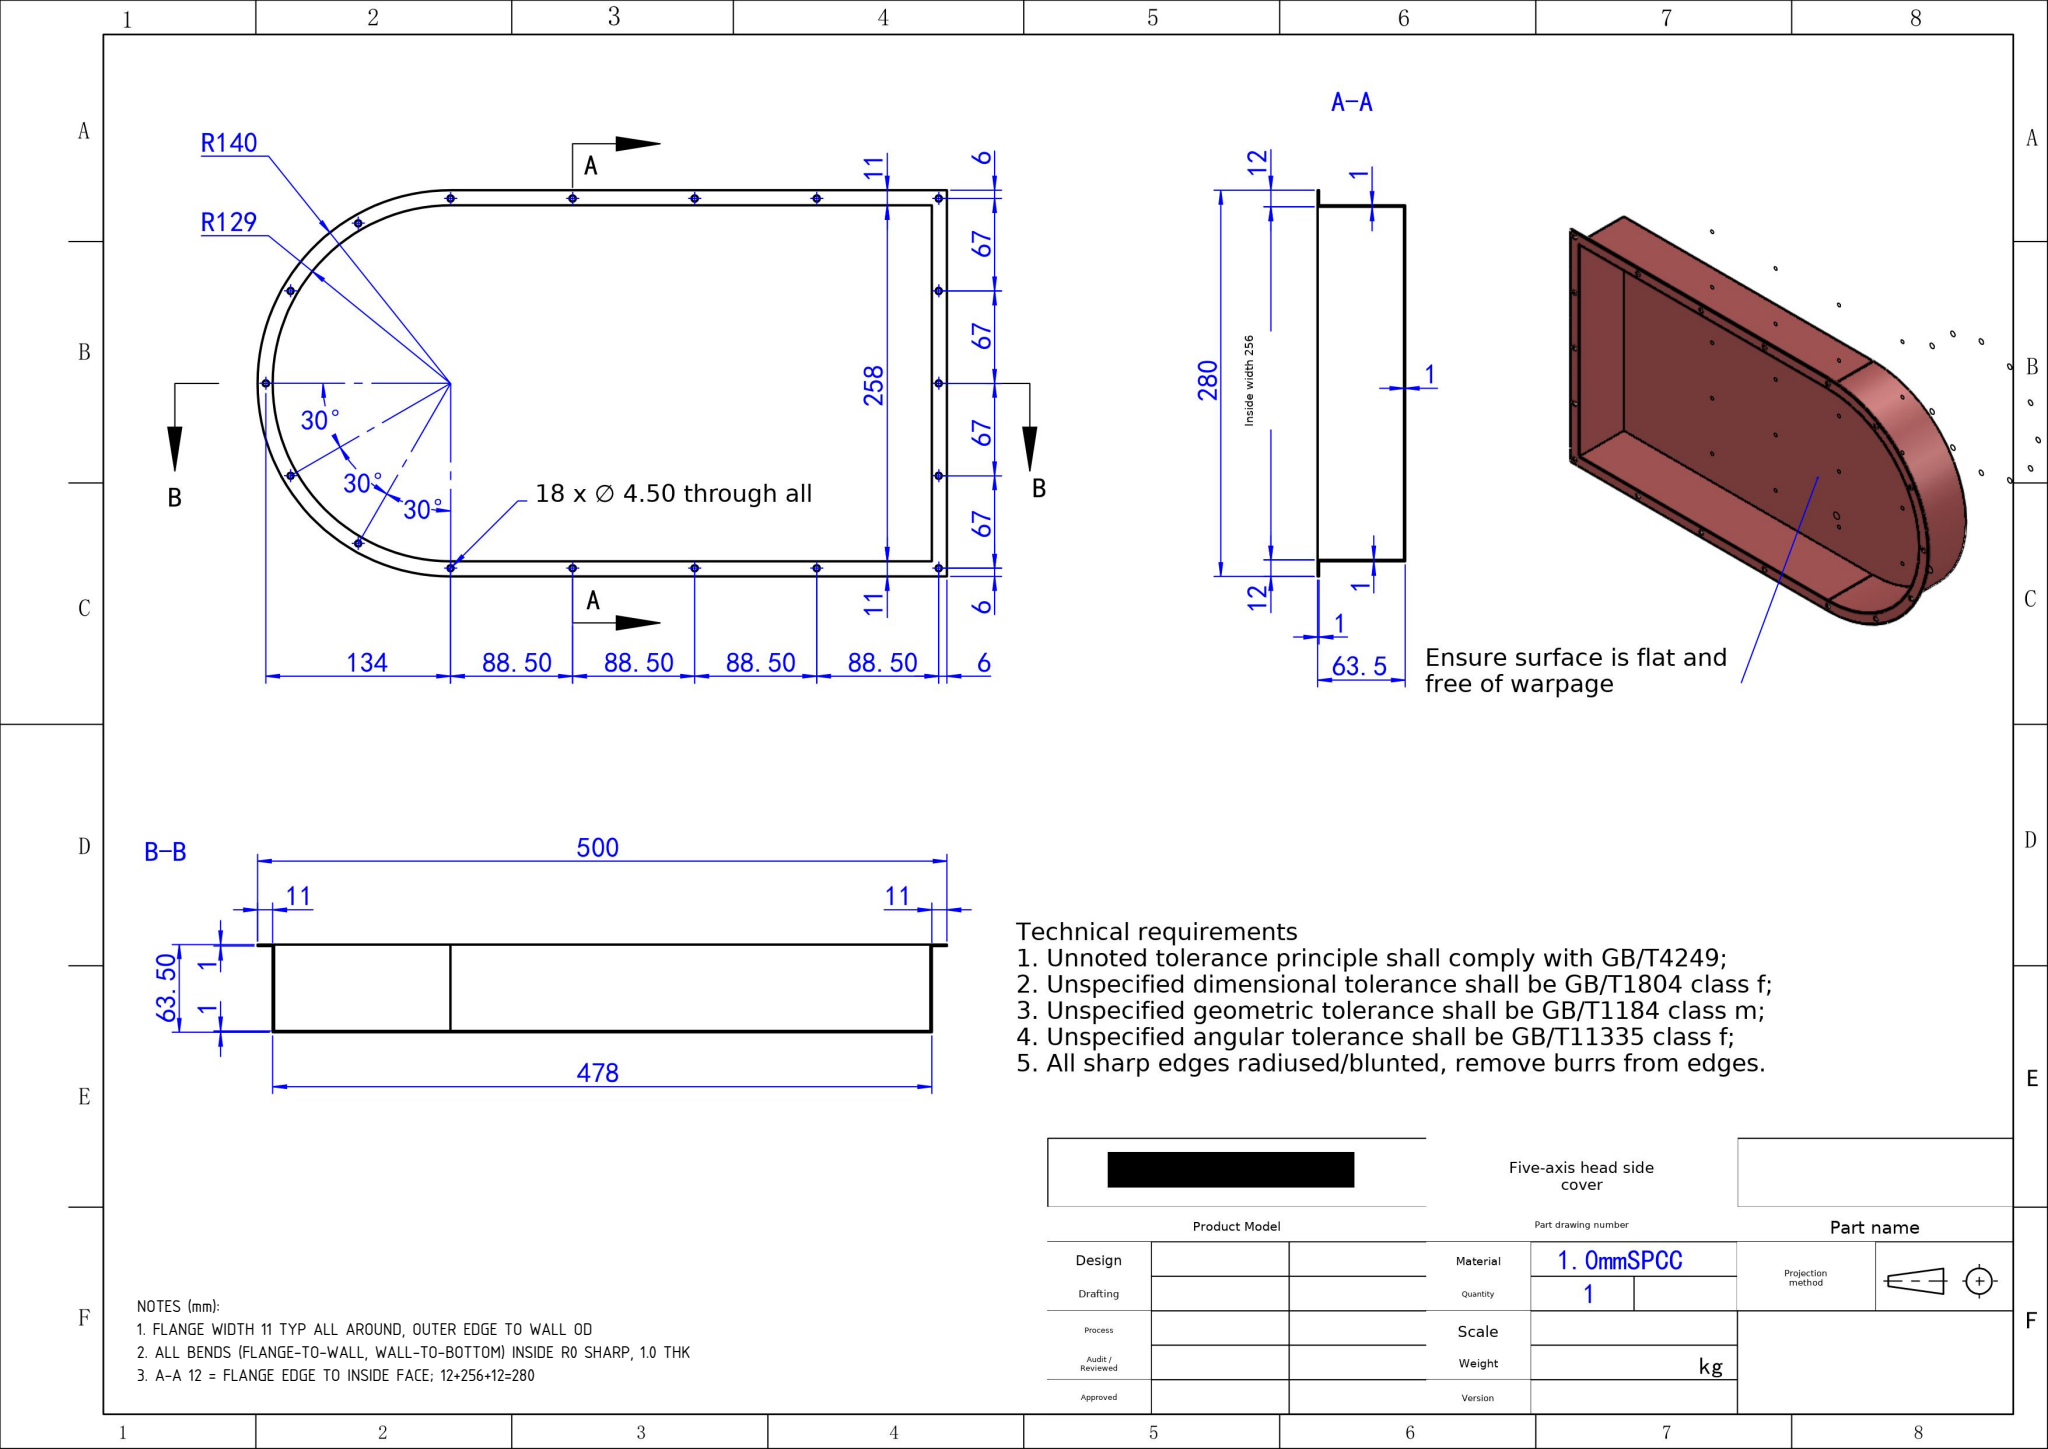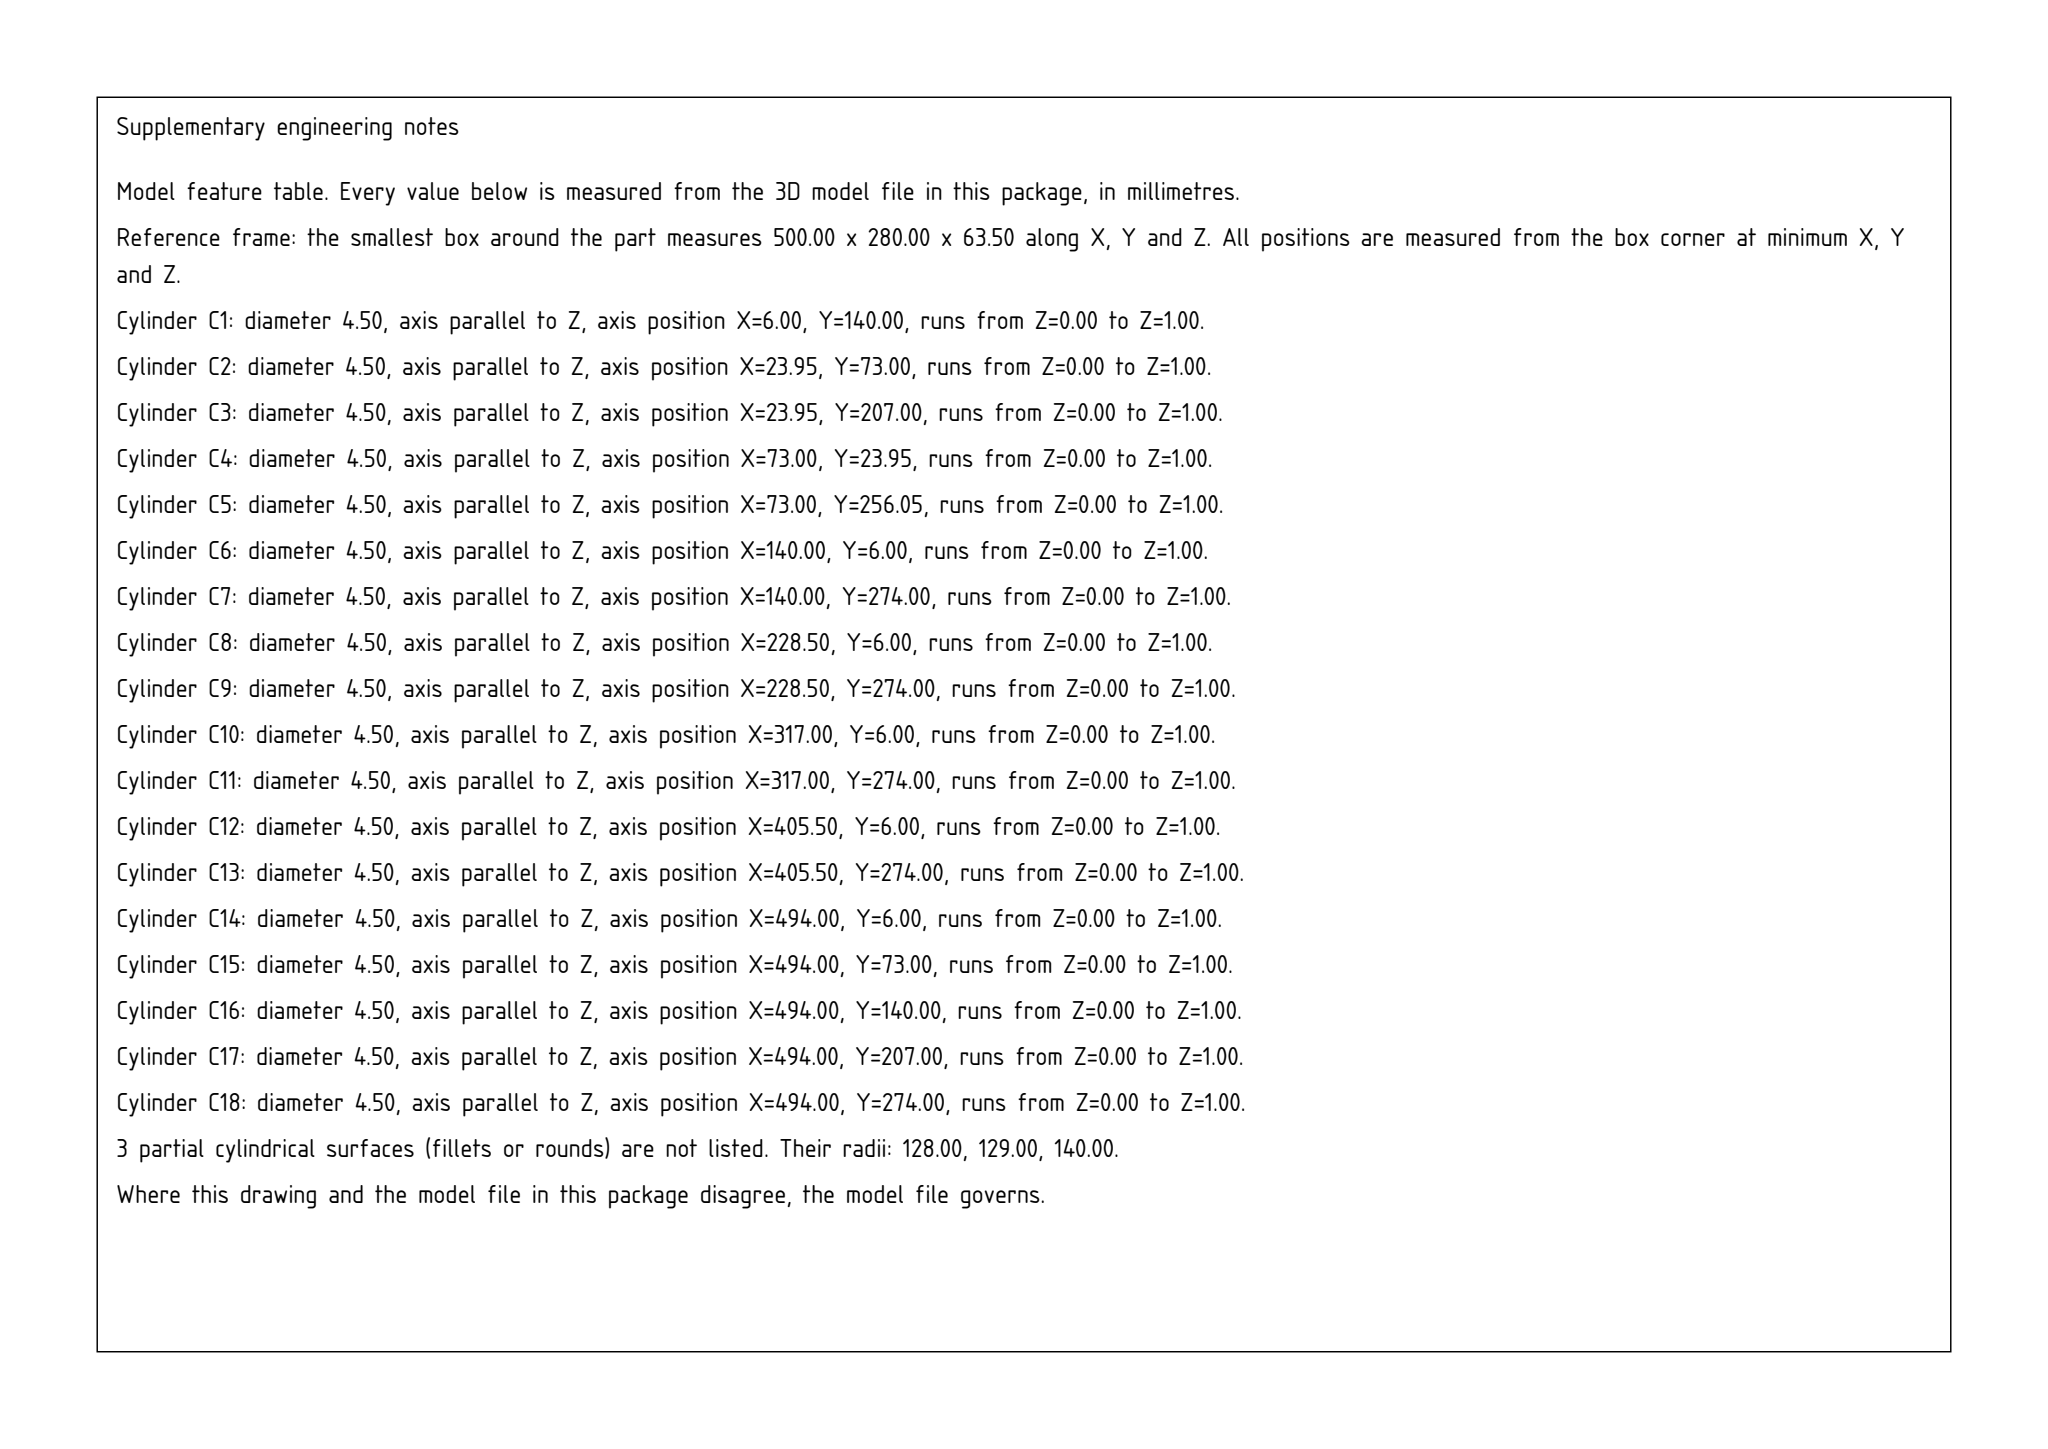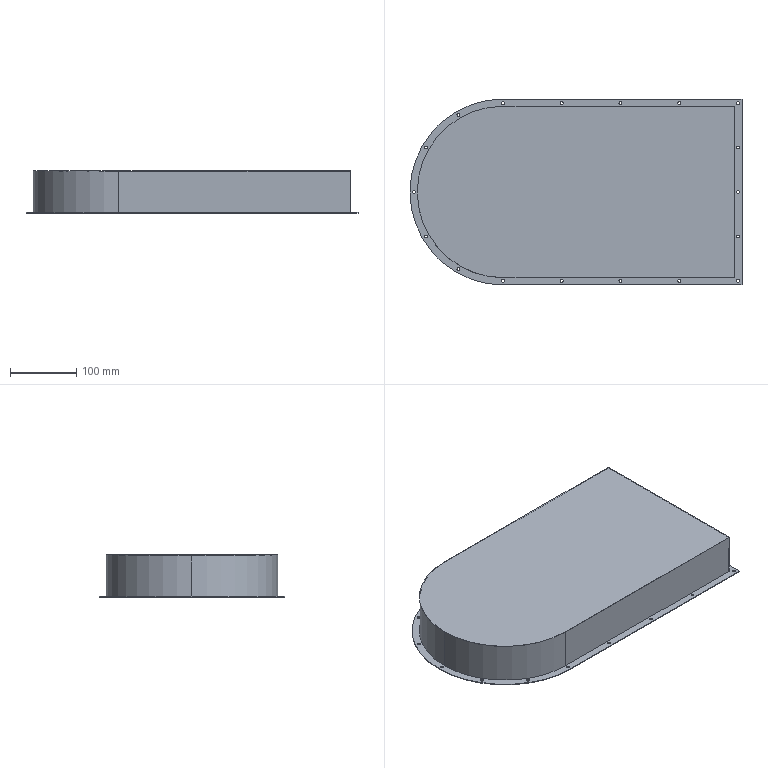Part | SolidWorks | mm | 1 solid | 53 faces | box 500 x 280 x 63.5 mm | volume 216157 mm3 | cylinder 40 | plane 13 | commonest cylinder face diameters 4.5 x36 258 x2 256 x1 280 x1
Drawing notes:
FLANGE WIDTH 11 TYP ALL AROUND, OUTER EDGE TO WALL OD | from the solid: Planes y=0/11, y=269/280, x=489/500; flange dia 280 vs wall OD dia 258 about (140,140)
ALL BENDS (FLANGE-TO-WALL, WALL-TO-BOTTOM) INSIDE R0 SHARP, 1.0 THK | from the solid: fillet_radii list empty; sharp 90 deg offset planes x488/489, y11/12, y268/269, z0/1, z62.5/63.5
A-A 12 = FLANGE EDGE TO INSIDE FACE; 12+256+12=280 | from the solid: Planes y=0,12,268,280; bbox Y=280